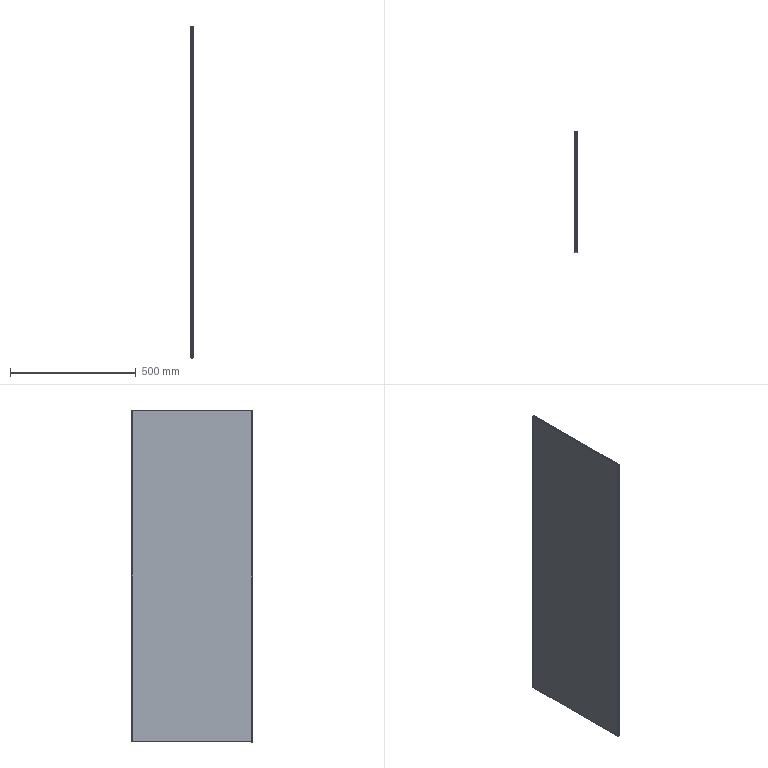Component | SolidWorks | LeftDoor-1 | 1 solid | 70 faces | volume 1031362 mm3 | plane 38 | spline 16 | cylinder 16 | commonest cylinder face diameters 5 x8 2 x8